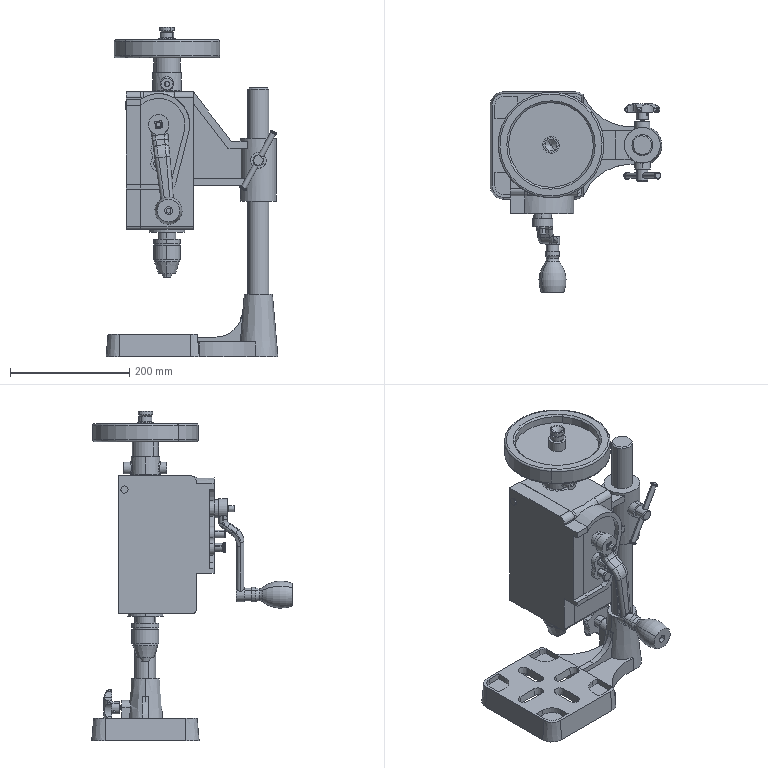Assembly | SolidWorks | mm | 18 component files | 20 solids | 657 faces | box 287.75 x 336 x 551.68 mm | volume 4042237 mm3 | cylinder 270 | plane 256 | cone 74 | torus 44 | spline 13 | commonest cylinder face diameters 20 x24 12 x21 4 x19 13 x18 8 x18 16 x14 26 x12 30 x11
Bill of materials:
11 | 1 |  | Thin, roughly rectangular, tray-like plate. One face has a pocket with a raised rim around it. One edge has two protruding tabs, and there is a small hole near one corner.
12 | 1 |  | Long, slender, stepped round shaft. It has a small-diameter tip at one end, a long main body with a slight circumferential break partway along, and a larger-diameter section at the other end.
13 | 1 |  | Axially symmetric stepped body. A short hollow tube is on top, above a larger cylindrical body with a shallow circumferential groove. Below that, a conical taper ends in a smaller conical tip.
18 | 1 |  | Solid cylindrical pin with chamfered ends and one round-bottomed circumferential groove placed off-center along its length.
1New | 1 |  | Bracket with a square, rounded-corner plate pierced by four slots in a cross pattern. A tapered arm with concave sides runs from the plate to a tapered hollow cylindrical boss that rises above the plate.
20 | 1 |  | Stepped cylindrical pin with a thin flanged head at one end, a reduced neck behind the head, a wider body section, and a slightly smaller-diameter remaining section with a chamfered end.
2 | 1 |  | Plain, solid, straight cylindrical rod with flat ends.
23 | 1 |  | Shaft with a short, small-diameter cylindrical spigot, a square prismatic block section, and a long cylindrical section of larger diameter than the spigot. The ends are chamfered.
25 | 1 |  | Funnel- or cup-shaped head with a conical recess and a small central through hole. Under the head are a chamfer, a short collar, a section with flats, and a small cylindrical stem with a chamfered end.
29 | 1 |  | Stepped cylindrical bushing: a smaller upper cylinder joined to a larger lower cylinder by a short reduced neck. It has a stepped through bore with a conical transition and a chamfered bottom edge.
3 | 1 |  | Shallow round disc or cap with a recessed top face inside a raised rim, a small central through hole, and a short cylindrical hub on the underside.
31 | 1 |  | Six-lobed star-shaped knob with a curved, domed profile and a rear cylindrical hub. The hub has a central bore and a small radial cross hole.
32 | 1 |  | Solid cylindrical pin: one long plain section and one short end section, separated by a groove with a rounded (concave) profile. The short end has a chamfer.
4 | 1 |  | T-shaped shape made of cylinders: a cylindrical hub, a long cross rod passing through it at right angles, and a stepped, chamfered stub shaft coming out of the hub along a third direction. Each end of the cross rod has a larger rounded cap like a flange.
5 | 1 |  | Lever or crank arm with an offset (joggle). One end has a larger round boss with a square through-hole. The other end has a smaller round boss with a small round through-hole. The arm bends sideways near the larger boss, so the two bosses sit in different planes.
6 | 1 |  | Solid stepped cylinder: a short cylinder with a larger diameter (head) joined to a longer plain cylindrical shank of smaller diameter on the same axis. Both ends are flat.
7 | 1 |  | Solid of revolution like a knob or finial. It has a bulbous, egg-shaped body with a flat large end, narrows to a concave neck, and ends in a two-step cylindrical spigot. A central round bore opens in the flat large end.
8 | 1 |  | Complex bracket-type body. It has a rectangular main block with a vertical cylindrical boss and bore, and an arm that slopes or steps out to a separate vertical ring boss with a large bore. Small cross-drilled lugs sit on the bosses. A curved side plate on the block carries several small holes, and there are thin flange or tab features.
Mates:
1. concentric | 1New-1 face at (17.957, 380.991, 189.093) dir (0, 0, 1) r 17.5 | 2-1 face at (17.957, 380.991, 777.093) dir (0, 0, -1) r 17.5
2. coincident | 1New-1 face at (17.957, 380.991, 327.093) dir (0, 0, -1) | 2-1 face at (17.957, 380.991, 327.093) dir (0, 0, -1)
3. concentric | 2-1 face at (17.957, 380.991, 777.093) dir (0, 0, -1) r 17.5 | 8-2 face at (17.957, 380.991, 692.751) dir (0, 0, -1) r 17.5
4. concentric | 4-1 face at (17.957, 363.491, 655.751) dir (0, -1, 0) r 5.4 | 8-2 face at (17.957, 340.991, 655.751) dir (0, -1, 0) r 5.4
5. coincident | 4-1 face at (17.957, 340.991, 655.751) dir (0, 1, 0) | 8-2 face at (17.957, 340.991, 655.751) dir (0, -1, 0)
6. concentric | 31-1 edge at (17.957, 424.991, 382.093) dir (0, -1, 0) r 5 | 32-1 face at (17.957, 432.991, 382.093) dir (0, -1, 0) r 5
7. coincident | 31-1 edge at (17.957, 424.991, 382.093) dir (0, -1, 0) r 5 | 32-1 edge at (17.957, 424.991, 382.093) dir (0, 1, 0) r 5
8. concentric | 5-1 face at (-132.516, 228.991, 571.696) dir (0, -1, 0) r 4 | 7-1 face at (-132.516, 214.991, 571.696) dir (0, 1, 0) r 4
9. coincident | 5-1 face at (-132.516, 214.991, 571.696) dir (0, -1, 0) | 7-1 face at (-132.516, 214.991, 571.696) dir (0, 1, 0)
10. coincident | 23-1 face at (-149.727, 265.991, 721.712) dir (-0.114, 0, 0.9935) | 5-1 face at (-149.727, 257.991, 721.712) dir (0.114, 0, -0.9935)
11. coincident | 23-1 face at (-143.082, 265.991, 716.435) dir (0.9935, 0, 0.114) | 5-1 face at (-143.082, 257.991, 716.435) dir (-0.9935, 0, -0.114)
12. coincident | 23-1 face at (-149.955, 243.991, 723.699) dir (0, -1, 0) | 5-1 face at (-149.043, 243.991, 715.751) dir (0, -1, 0)
13. concentric | 23-1 face at (-149.043, 231.091, 715.751) dir (0, -1, 0) r 6.5 | 8-2 face at (-149.043, 362.991, 715.751) dir (0, -1, 0) r 6.5
14. coincident | 5-1 face at (-149.043, 265.991, 715.751) dir (0, 1, 0) | 8-2 face at (17.957, 265.991, 655.751) dir (0, -1, 0)
15. coincident | 3-1 face at (-135.043, 380.991, 802.751) dir (0, 0, -1) | 8-2 face at (-135.043, 380.991, 802.751) dir (0, 0, 1)
16. concentric | 3-1 face at (-135.043, 380.991, 802.751) dir (0, 0, 1) r 124.355 | 8-2 face at (-135.043, 380.991, 739.751) dir (0, 0, 1) r 12.5
17. concentric | 12-1 face at (-135.043, 380.991, 817.213) dir (0, 0, 1) r 10 | 8-2 face at (-135.043, 380.991, 498.751) dir (0, 0, 1) r 8
18. concentric | 12-1 face at (-135.043, 380.991, 817.213) dir (0, 0, 1) r 10 | 13-1 face at (-135.043, 380.991, 535.213) dir (0, 0, 1) r 8.75
19. coincident | 12-1 face at (-142.665, 387.464, 535.213) dir (0, 0, 1) | 13-1 face at (-135.043, 380.991, 535.213) dir (0, 0, 1)
20. coincident | 1New-1 face at (-155.043, 420.991, 327.093) dir (0, 1, 0) | 32-1 edge at (17.957, 420.991, 382.093) dir (0, -1, 0) r 5
21. parallel | 8-2 face at (-110.361, 372.991, 770.751) dir (0, 0, 1) | 11-2 face at (-179.043, 368.991, 770.721) dir (0, 0, 1)
22. coincident | 8-2 face at (-179.043, 265.991, 655.751) dir (-1, 0, 0) | 11-2 edge at (-179.043, 305.988, 760.969) dir (1, 0, 0) r 10
23. concentric | 6-1 face at (-197.043, 415.991, 747.751) dir (-1, 0, 0) r 6 | 8-2 face at (-179.043, 415.991, 747.751) dir (-1, 0, 0) r 2.5
24. coincident | 6-1 edge at (-197.043, 415.991, 747.751) dir (1, 0, 0) r 6 | 11-2 face at (-197.043, 415.991, 747.751) dir (-1, 0, 0)
25. concentric | 6-1 edge at (-205.043, 415.991, 747.751) dir (1, 0, 0) r 6 | 11-2 edge at (-203.043, 415.991, 747.751) dir (-1, 0, 0) r 6
26. concentric | 20-1 face at (-149.043, 287.491, 650.751) dir (0, 1, 0) r 6.5 | 8-2 edge at (-149.043, 265.991, 650.751) dir (0, -1, 0) r 6.5
27. coincident | 20-1 edge at (-149.043, 265.991, 650.751) dir (0, 1, 0) r 6.5 | 8-2 face at (17.957, 265.991, 655.751) dir (0, -1, 0)
28. concentric | 18-1 face at (-149.043, 308.491, 673.144) dir (0, -1, 0) r 6.5 | 8-2 face at (-149.043, 305.991, 673.144) dir (0, -1, 0) r 6.5
29. coincident | 18-1 face at (-149.043, 247.491, 673.144) dir (0, -1, 0) | 20-1 face at (-149.043, 247.491, 650.751) dir (0, -1, 0)
30. concentric | 25-1 face at (-135.043, 380.991, 854.778) dir (0, 0, -1) r 12 | 3-1 face at (-135.043, 380.991, 802.751) dir (0, 0, 1) r 124.355
31. concentric | 25-1 face at (-135.043, 380.991, 854.778) dir (0, 0, -1) r 12 | 29-1 face at (-135.043, 380.991, 870.242) dir (0, 0, 1) r 8.5
32. coincident | 25-1 edge at (-135.043, 380.991, 854.778) dir (0, 0, -1) r 2.5 | 29-1 face at (-135.043, 380.991, 858.242) dir (0, 0, -1) r 1047.198
33. coincident | 29-1 edge at (-135.043, 380.991, 842.242) dir (0, 0, -1) r 13 | 3-1 face at (-135.043, 380.991, 842.242) dir (0, 0, 1)
34. concentric | 1New-1 face at (17.957, 397.491, 382.093) dir (0, 1, 0) r 5 | 32-1 face at (17.957, 432.991, 382.093) dir (0, -1, 0) r 5